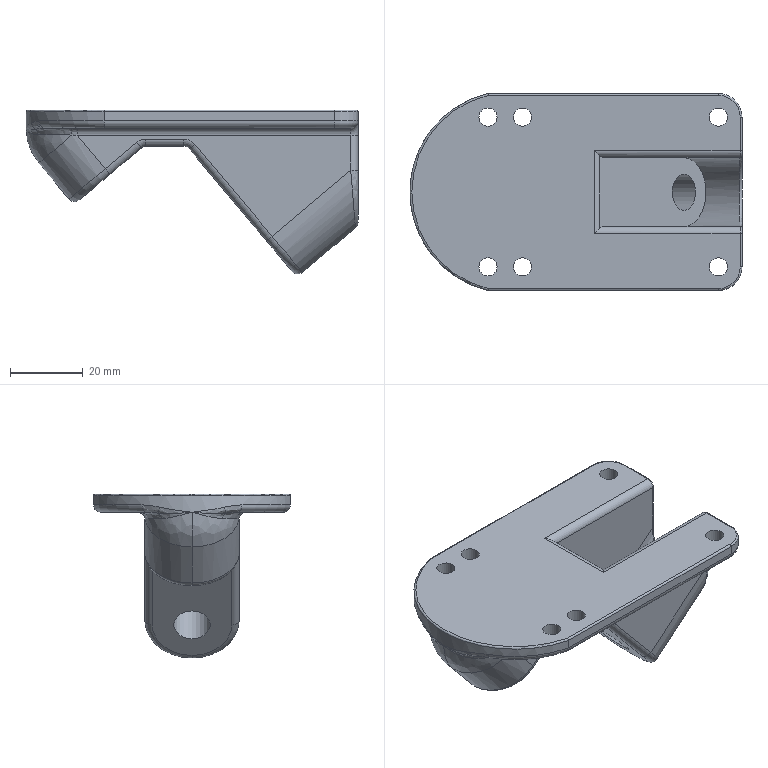Component | NX | BASEPLATE | 1 solid | 92 faces | volume 45434 mm3 | cylinder 41 | torus 19 | spline 17 | plane 14 | sphere 1 | commonest cylinder face diameters 4 x19 5 x6 1 x6 26 x4 13 x2 55.753 x1 10 x1 16 x1